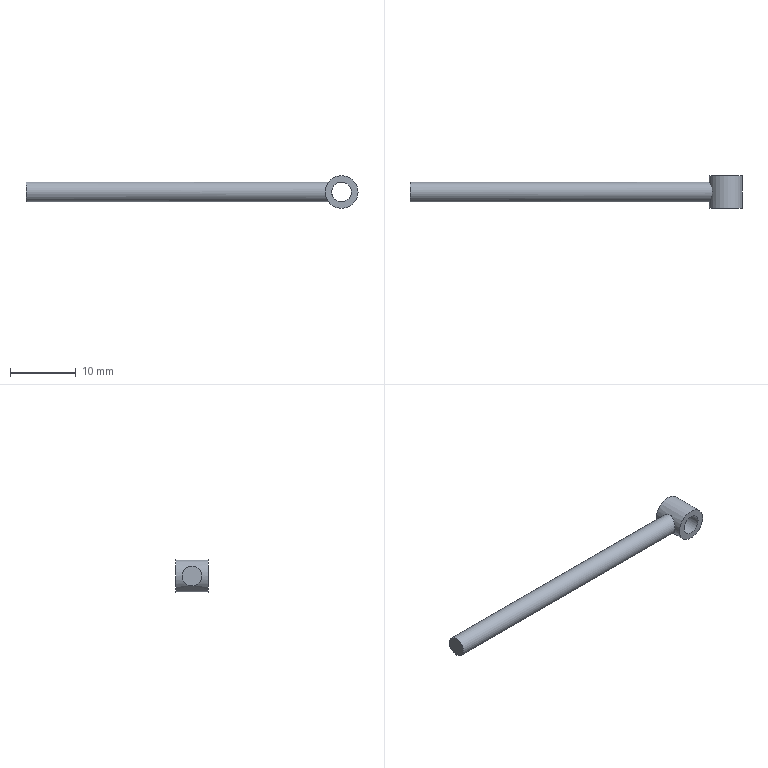Component | NX | LINK_6 | 1 solid | 6 faces | volume 385 mm3 | cylinder 3 | plane 3 | commonest cylinder face diameters 3 x2 5 x1